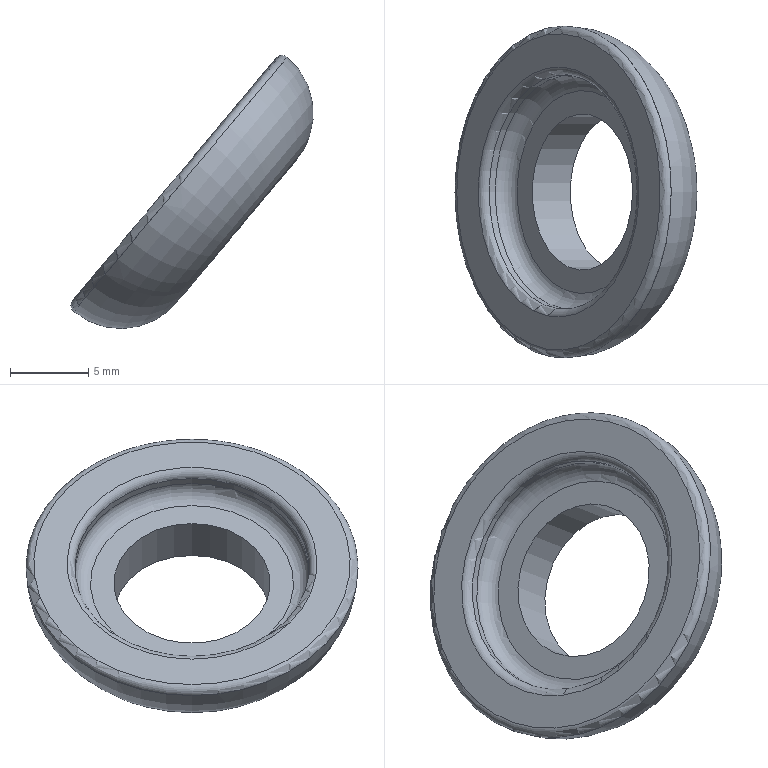Component | NX | HANGERWASHER_2 | 1 solid | 10 faces | box 15.51 x 21.25 x 17.49 mm | volume 954 mm3 | torus 4 | plane 3 | cylinder 3 | commonest cylinder face diameters 15 x1 21.25 x1 10 x1
STEP:
#1=CARTESIAN_POINT('',(0.,0.,0.));
#2=DIRECTION('',(0.,0.,1.));
#3=DIRECTION('',(1.,0.,0.));
#4=AXIS2_PLACEMENT_3D('',#1,#2,#3);
#5=CARTESIAN_POINT('',(452.874,0.,-59.196));
#6=VERTEX_POINT('',#5);
#7=CARTESIAN_POINT('',(449.66,0.,-63.026));
#8=DIRECTION('',(-0.766,0.,0.6428));
#9=DIRECTION('',(0.6428,0.,0.766));
#10=AXIS2_PLACEMENT_3D('',#7,#8,#9);
#11=CIRCLE('',#10,5.);
#12=CARTESIAN_POINT('',(449.66,0.,-63.026));
#13=DIRECTION('',(0.766,0.,-0.6428));
#14=DIRECTION('',(-0.6428,0.,-0.766));
#15=AXIS2_PLACEMENT_3D('',#12,#13,#14);
#16=PLANE('',#15);
#17=CARTESIAN_POINT('',(-5.,0.));
#18=CARTESIAN_POINT('',(-5.,8.66));
#19=CARTESIAN_POINT('',(2.5,4.33));
#20=CARTESIAN_POINT('',(10.,0.));
#21=CARTESIAN_POINT('',(2.5,-4.33));
#22=CARTESIAN_POINT('',(-5.,-8.66));
#23=CARTESIAN_POINT('',(-5.,0.));
#24=(BOUNDED_CURVE()B_SPLINE_CURVE(2,(#17,#18,#19,#20,#21,#22,#23),.UNSPECIFIED.,.T.,.F.)B_SPLINE_CURVE_WITH_KNOTS((1,2,2,2,2,1),(-2.094,0.,2.094,4.189,6.283,8.378),.UNSPECIFIED.)CURVE()GEOMETRIC_REPRESENTATION_ITEM()RATIONAL_B_SPLINE_CURVE((1.,0.5,1.,0.5,1.,0.5,1.))REPRESENTATION_ITEM(''));
#25=(GEOMETRIC_REPRESENTATION_CONTEXT(2)PARAMETRIC_REPRESENTATION_CONTEXT()REPRESENTATION_CONTEXT('',''));
#26=DEFINITIONAL_REPRESENTATION('',(#24),#25);
#27=PCURVE('',#16,#26);
#28=CARTESIAN_POINT('',(449.66,0.,-63.026));
#29=DIRECTION('',(-0.766,0.,0.6428));
#30=DIRECTION('',(0.6428,0.,0.766));
#31=AXIS2_PLACEMENT_3D('',#28,#29,#30);
#32=CYLINDRICAL_SURFACE('',#31,5.);
#33=CARTESIAN_POINT('',(0.,0.));
#34=DIRECTION('',(1.,0.));
#35=VECTOR('',#34,1.);
#36=LINE('',#33,#35);
#37=(GEOMETRIC_REPRESENTATION_CONTEXT(2)PARAMETRIC_REPRESENTATION_CONTEXT()REPRESENTATION_CONTEXT('',''));
#38=DEFINITIONAL_REPRESENTATION('',(#36),#37);
#39=PCURVE('',#32,#38);
#40=SURFACE_CURVE('',#11,(#27,#39),.PCURVE_S1.);
#41=EDGE_CURVE('',#6,#6,#40,.T.);
#42=ORIENTED_EDGE('',*,*,#41,.T.);
#43=EDGE_LOOP('',(#42));
#44=FACE_BOUND('',#43,.T.);
#45=CARTESIAN_POINT('',(445.832,0.,-67.588));
#46=VERTEX_POINT('',#45);
#47=CARTESIAN_POINT('',(449.66,0.,-63.026));
#48=DIRECTION('',(0.766,0.,-0.6428));
#49=DIRECTION('',(-0.6428,0.,-0.766));
#50=AXIS2_PLACEMENT_3D('',#47,#48,#49);
#51=CIRCLE('',#50,5.955);
#52=CARTESIAN_POINT('',(0.,0.));
#53=DIRECTION('',(1.,0.));
#54=AXIS2_PLACEMENT_2D('',#52,#53);
#55=CIRCLE('',#54,5.955);
#56=(GEOMETRIC_REPRESENTATION_CONTEXT(2)PARAMETRIC_REPRESENTATION_CONTEXT()REPRESENTATION_CONTEXT('',''));
#57=DEFINITIONAL_REPRESENTATION('',(#55),#56);
#58=PCURVE('',#16,#57);
#59=CARTESIAN_POINT('',(446.083,0.,-60.025));
#60=DIRECTION('',(0.766,0.,-0.6428));
#61=DIRECTION('',(-0.6428,0.,-0.766));
#62=AXIS2_PLACEMENT_3D('',#59,#60,#61);
#63=TOROIDAL_SURFACE('',#62,5.955,4.67);
#64=CARTESIAN_POINT('',(0.,7.854));
#65=DIRECTION('',(1.,0.));
#66=VECTOR('',#65,1.);
#67=LINE('',#64,#66);
#68=(GEOMETRIC_REPRESENTATION_CONTEXT(2)PARAMETRIC_REPRESENTATION_CONTEXT()REPRESENTATION_CONTEXT('',''));
#69=DEFINITIONAL_REPRESENTATION('',(#67),#68);
#70=PCURVE('',#63,#69);
#71=SURFACE_CURVE('',#51,(#58,#70),.PCURVE_S1.);
#72=EDGE_CURVE('',#46,#46,#71,.T.);
#73=ORIENTED_EDGE('',*,*,#72,.T.);
#74=EDGE_LOOP('',(#73));
#75=FACE_BOUND('',#74,.T.);
#76=ADVANCED_FACE('',(#44,#75),#16,.T.);
#77=CARTESIAN_POINT('',(450.9,0.,-54.276));
#78=VERTEX_POINT('',#77);
#79=CARTESIAN_POINT('',(441.258,0.,-65.767));
#80=VERTEX_POINT('',#79);
#81=CARTESIAN_POINT('',(446.079,0.,-60.021));
#82=DIRECTION('',(-0.766,0.,0.6428));
#83=DIRECTION('',(-0.6428,0.,-0.766));
#84=AXIS2_PLACEMENT_3D('',#81,#82,#83);
#85=CIRCLE('',#84,7.5);
#86=CARTESIAN_POINT('',(449.66,0.,-63.026));
#87=DIRECTION('',(-0.766,0.,0.6428));
#88=DIRECTION('',(0.6428,0.,0.766));
#89=AXIS2_PLACEMENT_3D('',#86,#87,#88);
#90=CYLINDRICAL_SURFACE('',#89,7.5);
#91=CARTESIAN_POINT('',(-3.142,4.675));
#92=DIRECTION('',(1.,0.));
#93=VECTOR('',#92,1.);
#94=LINE('',#91,#93);
#95=(GEOMETRIC_REPRESENTATION_CONTEXT(2)PARAMETRIC_REPRESENTATION_CONTEXT()REPRESENTATION_CONTEXT('',''));
#96=DEFINITIONAL_REPRESENTATION('',(#94),#95);
#97=PCURVE('',#90,#96);
#98=CARTESIAN_POINT('',(446.079,0.,-60.021));
#99=DIRECTION('',(0.766,0.,-0.6428));
#100=DIRECTION('',(-0.6428,0.,-0.766));
#101=AXIS2_PLACEMENT_3D('',#98,#99,#100);
#102=TOROIDAL_SURFACE('',#101,8.,0.5);
#103=CARTESIAN_POINT('',(6.283,3.142));
#104=DIRECTION('',(-1.,0.));
#105=VECTOR('',#104,1.);
#106=LINE('',#103,#105);
#107=(GEOMETRIC_REPRESENTATION_CONTEXT(2)PARAMETRIC_REPRESENTATION_CONTEXT()REPRESENTATION_CONTEXT('',''));
#108=DEFINITIONAL_REPRESENTATION('',(#106),#107);
#109=PCURVE('',#102,#108);
#110=SURFACE_CURVE('',#85,(#97,#109),.PCURVE_S1.);
#111=EDGE_CURVE('',#78,#80,#110,.T.);
#112=ORIENTED_EDGE('',*,*,#111,.F.);
#113=CARTESIAN_POINT('',(451.283,0.,-54.597));
#114=VERTEX_POINT('',#113);
#115=CARTESIAN_POINT('',(451.283,-0.,-54.597));
#116=CARTESIAN_POINT('',(450.9,-0.,-54.276));
#117=B_SPLINE_CURVE_WITH_KNOTS('',1,(#115,#116),.UNSPECIFIED.,.F.,.F.,(2,2),(4.175,4.675),.PIECEWISE_BEZIER_KNOTS.);
#118=CARTESIAN_POINT('',(0.,0.));
#119=DIRECTION('',(0.,1.));
#120=VECTOR('',#119,1.);
#121=LINE('',#118,#120);
#122=(GEOMETRIC_REPRESENTATION_CONTEXT(2)PARAMETRIC_REPRESENTATION_CONTEXT()REPRESENTATION_CONTEXT('',''));
#123=DEFINITIONAL_REPRESENTATION('',(#121),#122);
#124=PCURVE('',#90,#123);
#125=CARTESIAN_POINT('',(6.283,0.));
#126=DIRECTION('',(0.,1.));
#127=VECTOR('',#126,1.);
#128=LINE('',#125,#127);
#129=(GEOMETRIC_REPRESENTATION_CONTEXT(2)PARAMETRIC_REPRESENTATION_CONTEXT()REPRESENTATION_CONTEXT('',''));
#130=DEFINITIONAL_REPRESENTATION('',(#128),#129);
#131=PCURVE('',#90,#130);
#132=SEAM_CURVE('',#117,(#124,#131),.PCURVE_S1.);
#133=EDGE_CURVE('',#114,#78,#132,.T.);
#134=ORIENTED_EDGE('',*,*,#133,.F.);
#135=CARTESIAN_POINT('',(446.462,0.,-60.343));
#136=DIRECTION('',(0.766,0.,-0.6428));
#137=DIRECTION('',(0.6428,0.,0.766));
#138=AXIS2_PLACEMENT_3D('',#135,#136,#137);
#139=CIRCLE('',#138,7.5);
#140=CARTESIAN_POINT('',(6.283,4.175));
#141=DIRECTION('',(-1.,0.));
#142=VECTOR('',#141,1.);
#143=LINE('',#140,#142);
#144=(GEOMETRIC_REPRESENTATION_CONTEXT(2)PARAMETRIC_REPRESENTATION_CONTEXT()REPRESENTATION_CONTEXT('',''));
#145=DEFINITIONAL_REPRESENTATION('',(#143),#144);
#146=PCURVE('',#90,#145);
#147=CARTESIAN_POINT('',(446.462,0.,-60.343));
#148=DIRECTION('',(-0.766,0.,0.6428));
#149=DIRECTION('',(0.6428,0.,0.766));
#150=AXIS2_PLACEMENT_3D('',#147,#148,#149);
#151=TOROIDAL_SURFACE('',#150,6.5,1.);
#152=CARTESIAN_POINT('',(6.283,6.283));
#153=DIRECTION('',(-1.,0.));
#154=VECTOR('',#153,1.);
#155=LINE('',#152,#154);
#156=(GEOMETRIC_REPRESENTATION_CONTEXT(2)PARAMETRIC_REPRESENTATION_CONTEXT()REPRESENTATION_CONTEXT('',''));
#157=DEFINITIONAL_REPRESENTATION('',(#155),#156);
#158=PCURVE('',#151,#157);
#159=SURFACE_CURVE('',#139,(#146,#158),.PCURVE_S1.);
#160=EDGE_CURVE('',#114,#114,#159,.T.);
#161=ORIENTED_EDGE('',*,*,#160,.F.);
#162=ORIENTED_EDGE('',*,*,#133,.T.);
#163=CARTESIAN_POINT('',(446.079,0.,-60.021));
#164=DIRECTION('',(-0.766,0.,0.6428));
#165=DIRECTION('',(-0.6428,0.,-0.766));
#166=AXIS2_PLACEMENT_3D('',#163,#164,#165);
#167=CIRCLE('',#166,7.5);
#168=CARTESIAN_POINT('',(3.142,4.675));
#169=DIRECTION('',(1.,0.));
#170=VECTOR('',#169,1.);
#171=LINE('',#168,#170);
#172=(GEOMETRIC_REPRESENTATION_CONTEXT(2)PARAMETRIC_REPRESENTATION_CONTEXT()REPRESENTATION_CONTEXT('',''));
#173=DEFINITIONAL_REPRESENTATION('',(#171),#172);
#174=PCURVE('',#90,#173);
#175=CARTESIAN_POINT('',(6.283,3.142));
#176=DIRECTION('',(-1.,-0.));
#177=VECTOR('',#176,1.);
#178=LINE('',#175,#177);
#179=(GEOMETRIC_REPRESENTATION_CONTEXT(2)PARAMETRIC_REPRESENTATION_CONTEXT()REPRESENTATION_CONTEXT('',''));
#180=DEFINITIONAL_REPRESENTATION('',(#178),#179);
#181=PCURVE('',#102,#180);
#182=SURFACE_CURVE('',#167,(#174,#181),.PCURVE_S1.);
#183=EDGE_CURVE('',#80,#78,#182,.T.);
#184=ORIENTED_EDGE('',*,*,#183,.F.);
#185=EDGE_LOOP('',(#112,#134,#161,#162,#184));
#186=FACE_BOUND('',#185,.F.);
#187=ADVANCED_FACE('',(#186),#90,.F.);
#188=CARTESIAN_POINT('',(439.249,0.,-68.161));
#189=VERTEX_POINT('',#188);
#190=CARTESIAN_POINT('',(446.079,0.,-60.021));
#191=DIRECTION('',(0.766,0.,-0.6428));
#192=DIRECTION('',(-0.6428,0.,-0.766));
#193=AXIS2_PLACEMENT_3D('',#190,#191,#192);
#194=CIRCLE('',#193,10.625);
#195=CARTESIAN_POINT('',(449.66,0.,-63.026));
#196=DIRECTION('',(-0.766,0.,0.6428));
#197=DIRECTION('',(0.6428,0.,0.766));
#198=AXIS2_PLACEMENT_3D('',#195,#196,#197);
#199=CYLINDRICAL_SURFACE('',#198,10.625);
#200=CARTESIAN_POINT('',(9.425,4.675));
#201=DIRECTION('',(-1.,0.));
#202=VECTOR('',#201,1.);
#203=LINE('',#200,#202);
#204=(GEOMETRIC_REPRESENTATION_CONTEXT(2)PARAMETRIC_REPRESENTATION_CONTEXT()REPRESENTATION_CONTEXT('',''));
#205=DEFINITIONAL_REPRESENTATION('',(#203),#204);
#206=PCURVE('',#199,#205);
#207=CARTESIAN_POINT('',(446.079,0.,-60.021));
#208=DIRECTION('',(0.766,0.,-0.6428));
#209=DIRECTION('',(-0.6428,0.,-0.766));
#210=AXIS2_PLACEMENT_3D('',#207,#208,#209);
#211=TOROIDAL_SURFACE('',#210,10.125,0.5);
#212=CARTESIAN_POINT('',(0.,6.283));
#213=DIRECTION('',(1.,0.));
#214=VECTOR('',#213,1.);
#215=LINE('',#212,#214);
#216=(GEOMETRIC_REPRESENTATION_CONTEXT(2)PARAMETRIC_REPRESENTATION_CONTEXT()REPRESENTATION_CONTEXT('',''));
#217=DEFINITIONAL_REPRESENTATION('',(#215),#216);
#218=PCURVE('',#211,#217);
#219=SURFACE_CURVE('',#194,(#206,#218),.PCURVE_S1.);
#220=EDGE_CURVE('',#189,#189,#219,.T.);
#221=ORIENTED_EDGE('',*,*,#220,.T.);
#222=CARTESIAN_POINT('',(439.253,0.,-68.164));
#223=VERTEX_POINT('',#222);
#224=CARTESIAN_POINT('',(439.253,0.,-68.164));
#225=CARTESIAN_POINT('',(439.249,0.,-68.161));
#226=B_SPLINE_CURVE_WITH_KNOTS('',1,(#224,#225),.UNSPECIFIED.,.F.,.F.,(2,2),(4.67,4.675),.PIECEWISE_BEZIER_KNOTS.);
#227=CARTESIAN_POINT('',(3.142,0.));
#228=DIRECTION('',(0.,1.));
#229=VECTOR('',#228,1.);
#230=LINE('',#227,#229);
#231=(GEOMETRIC_REPRESENTATION_CONTEXT(2)PARAMETRIC_REPRESENTATION_CONTEXT()REPRESENTATION_CONTEXT('',''));
#232=DEFINITIONAL_REPRESENTATION('',(#230),#231);
#233=PCURVE('',#199,#232);
#234=CARTESIAN_POINT('',(9.425,0.));
#235=DIRECTION('',(0.,1.));
#236=VECTOR('',#235,1.);
#237=LINE('',#234,#236);
#238=(GEOMETRIC_REPRESENTATION_CONTEXT(2)PARAMETRIC_REPRESENTATION_CONTEXT()REPRESENTATION_CONTEXT('',''));
#239=DEFINITIONAL_REPRESENTATION('',(#237),#238);
#240=PCURVE('',#199,#239);
#241=SEAM_CURVE('',#226,(#233,#240),.PCURVE_S1.);
#242=EDGE_CURVE('',#223,#189,#241,.T.);
#243=ORIENTED_EDGE('',*,*,#242,.F.);
#244=CARTESIAN_POINT('',(446.083,0.,-60.025));
#245=DIRECTION('',(-0.766,0.,0.6428));
#246=DIRECTION('',(-0.6428,0.,-0.766));
#247=AXIS2_PLACEMENT_3D('',#244,#245,#246);
#248=CIRCLE('',#247,10.625);
#249=CARTESIAN_POINT('',(3.142,4.67));
#250=DIRECTION('',(1.,0.));
#251=VECTOR('',#250,1.);
#252=LINE('',#249,#251);
#253=(GEOMETRIC_REPRESENTATION_CONTEXT(2)PARAMETRIC_REPRESENTATION_CONTEXT()REPRESENTATION_CONTEXT('',''));
#254=DEFINITIONAL_REPRESENTATION('',(#252),#253);
#255=PCURVE('',#199,#254);
#256=CARTESIAN_POINT('',(6.283,6.283));
#257=DIRECTION('',(-1.,0.));
#258=VECTOR('',#257,1.);
#259=LINE('',#256,#258);
#260=(GEOMETRIC_REPRESENTATION_CONTEXT(2)PARAMETRIC_REPRESENTATION_CONTEXT()REPRESENTATION_CONTEXT('',''));
#261=DEFINITIONAL_REPRESENTATION('',(#259),#260);
#262=PCURVE('',#63,#261);
#263=SURFACE_CURVE('',#248,(#255,#262),.PCURVE_S1.);
#264=EDGE_CURVE('',#223,#223,#263,.T.);
#265=ORIENTED_EDGE('',*,*,#264,.T.);
#266=ORIENTED_EDGE('',*,*,#242,.T.);
#267=EDGE_LOOP('',(#221,#243,#265,#266));
#268=FACE_BOUND('',#267,.T.);
#269=ADVANCED_FACE('',(#268),#199,.T.);
#270=CARTESIAN_POINT('',(439.188,0.,-67.456));
#271=VERTEX_POINT('',#270);
#272=CARTESIAN_POINT('',(445.696,0.,-59.7));
#273=DIRECTION('',(-0.766,0.,0.6428));
#274=DIRECTION('',(-0.6428,0.,-0.766));
#275=AXIS2_PLACEMENT_3D('',#272,#273,#274);
#276=CIRCLE('',#275,10.125);
#277=CARTESIAN_POINT('',(438.866,0.,-67.839));
#278=DIRECTION('',(0.766,0.,-0.6428));
#279=DIRECTION('',(-0.6428,0.,-0.766));
#280=AXIS2_PLACEMENT_3D('',#277,#278,#279);
#281=PLANE('',#280);
#282=CARTESIAN_POINT('',(-0.5,0.));
#283=CARTESIAN_POINT('',(-0.5,-17.537));
#284=CARTESIAN_POINT('',(-15.688,-8.769));
#285=CARTESIAN_POINT('',(-30.875,-0.));
#286=CARTESIAN_POINT('',(-15.688,8.769));
#287=CARTESIAN_POINT('',(-0.5,17.537));
#288=CARTESIAN_POINT('',(-0.5,0.));
#289=(BOUNDED_CURVE()B_SPLINE_CURVE(2,(#282,#283,#284,#285,#286,#287,#288),.UNSPECIFIED.,.T.,.F.)B_SPLINE_CURVE_WITH_KNOTS((1,2,2,2,2,1),(-2.094,0.,2.094,4.189,6.283,8.378),.UNSPECIFIED.)CURVE()GEOMETRIC_REPRESENTATION_ITEM()RATIONAL_B_SPLINE_CURVE((1.,0.5,1.,0.5,1.,0.5,1.))REPRESENTATION_ITEM(''));
#290=(GEOMETRIC_REPRESENTATION_CONTEXT(2)PARAMETRIC_REPRESENTATION_CONTEXT()REPRESENTATION_CONTEXT('',''));
#291=DEFINITIONAL_REPRESENTATION('',(#289),#290);
#292=PCURVE('',#281,#291);
#293=CARTESIAN_POINT('',(6.283,4.712));
#294=DIRECTION('',(-1.,0.));
#295=VECTOR('',#294,1.);
#296=LINE('',#293,#295);
#297=(GEOMETRIC_REPRESENTATION_CONTEXT(2)PARAMETRIC_REPRESENTATION_CONTEXT()REPRESENTATION_CONTEXT('',''));
#298=DEFINITIONAL_REPRESENTATION('',(#296),#297);
#299=PCURVE('',#211,#298);
#300=SURFACE_CURVE('',#276,(#292,#299),.PCURVE_S1.);
#301=EDGE_CURVE('',#271,#271,#300,.T.);
#302=ORIENTED_EDGE('',*,*,#301,.T.);
#303=EDGE_LOOP('',(#302));
#304=FACE_BOUND('',#303,.T.);
#305=CARTESIAN_POINT('',(440.554,0.,-65.828));
#306=VERTEX_POINT('',#305);
#307=CARTESIAN_POINT('',(445.696,0.,-59.7));
#308=DIRECTION('',(0.766,0.,-0.6428));
#309=DIRECTION('',(-0.6428,0.,-0.766));
#310=AXIS2_PLACEMENT_3D('',#307,#308,#309);
#311=CIRCLE('',#310,8.);
#312=CARTESIAN_POINT('',(-10.625,0.));
#313=DIRECTION('',(1.,0.));
#314=AXIS2_PLACEMENT_2D('',#312,#313);
#315=CIRCLE('',#314,8.);
#316=(GEOMETRIC_REPRESENTATION_CONTEXT(2)PARAMETRIC_REPRESENTATION_CONTEXT()REPRESENTATION_CONTEXT('',''));
#317=DEFINITIONAL_REPRESENTATION('',(#315),#316);
#318=PCURVE('',#281,#317);
#319=CARTESIAN_POINT('',(0.,4.712));
#320=DIRECTION('',(1.,0.));
#321=VECTOR('',#320,1.);
#322=LINE('',#319,#321);
#323=(GEOMETRIC_REPRESENTATION_CONTEXT(2)PARAMETRIC_REPRESENTATION_CONTEXT()REPRESENTATION_CONTEXT('',''));
#324=DEFINITIONAL_REPRESENTATION('',(#322),#323);
#325=PCURVE('',#102,#324);
#326=SURFACE_CURVE('',#311,(#318,#325),.PCURVE_S1.);
#327=EDGE_CURVE('',#306,#306,#326,.T.);
#328=ORIENTED_EDGE('',*,*,#327,.T.);
#329=EDGE_LOOP('',(#328));
#330=FACE_BOUND('',#329,.T.);
#331=ADVANCED_FACE('',(#304,#330),#281,.F.);
#332=CARTESIAN_POINT('',(450.442,0.,-57.155));
#333=VERTEX_POINT('',#332);
#334=CARTESIAN_POINT('',(447.228,0.,-60.986));
#335=DIRECTION('',(-0.766,0.,0.6428));
#336=DIRECTION('',(0.6428,0.,0.766));
#337=AXIS2_PLACEMENT_3D('',#334,#335,#336);
#338=CIRCLE('',#337,5.);
#339=CARTESIAN_POINT('',(447.228,0.,-60.986));
#340=DIRECTION('',(-0.766,0.,0.6428));
#341=DIRECTION('',(0.6428,0.,0.766));
#342=AXIS2_PLACEMENT_3D('',#339,#340,#341);
#343=PLANE('',#342);
#344=CARTESIAN_POINT('',(0.,0.));
#345=DIRECTION('',(1.,0.));
#346=AXIS2_PLACEMENT_2D('',#344,#345);
#347=CIRCLE('',#346,5.);
#348=(GEOMETRIC_REPRESENTATION_CONTEXT(2)PARAMETRIC_REPRESENTATION_CONTEXT()REPRESENTATION_CONTEXT('',''));
#349=DEFINITIONAL_REPRESENTATION('',(#347),#348);
#350=PCURVE('',#343,#349);
#351=CARTESIAN_POINT('',(0.,3.175));
#352=DIRECTION('',(1.,0.));
#353=VECTOR('',#352,1.);
#354=LINE('',#351,#353);
#355=(GEOMETRIC_REPRESENTATION_CONTEXT(2)PARAMETRIC_REPRESENTATION_CONTEXT()REPRESENTATION_CONTEXT('',''));
#356=DEFINITIONAL_REPRESENTATION('',(#354),#355);
#357=PCURVE('',#32,#356);
#358=SURFACE_CURVE('',#338,(#350,#357),.PCURVE_S1.);
#359=EDGE_CURVE('',#333,#333,#358,.T.);
#360=ORIENTED_EDGE('',*,*,#359,.F.);
#361=EDGE_LOOP('',(#360));
#362=FACE_BOUND('',#361,.T.);
#363=CARTESIAN_POINT('',(451.406,0.,-56.006));
#364=VERTEX_POINT('',#363);
#365=CARTESIAN_POINT('',(447.228,0.,-60.986));
#366=DIRECTION('',(-0.766,0.,0.6428));
#367=DIRECTION('',(0.6428,0.,0.766));
#368=AXIS2_PLACEMENT_3D('',#365,#366,#367);
#369=CIRCLE('',#368,6.5);
#370=CARTESIAN_POINT('',(0.,0.));
#371=DIRECTION('',(1.,0.));
#372=AXIS2_PLACEMENT_2D('',#370,#371);
#373=CIRCLE('',#372,6.5);
#374=(GEOMETRIC_REPRESENTATION_CONTEXT(2)PARAMETRIC_REPRESENTATION_CONTEXT()REPRESENTATION_CONTEXT('',''));
#375=DEFINITIONAL_REPRESENTATION('',(#373),#374);
#376=PCURVE('',#343,#375);
#377=CARTESIAN_POINT('',(0.,4.712));
#378=DIRECTION('',(1.,0.));
#379=VECTOR('',#378,1.);
#380=LINE('',#377,#379);
#381=(GEOMETRIC_REPRESENTATION_CONTEXT(2)PARAMETRIC_REPRESENTATION_CONTEXT()REPRESENTATION_CONTEXT('',''));
#382=DEFINITIONAL_REPRESENTATION('',(#380),#381);
#383=PCURVE('',#151,#382);
#384=SURFACE_CURVE('',#369,(#376,#383),.PCURVE_S1.);
#385=EDGE_CURVE('',#364,#364,#384,.T.);
#386=ORIENTED_EDGE('',*,*,#385,.T.);
#387=EDGE_LOOP('',(#386));
#388=FACE_BOUND('',#387,.T.);
#389=ADVANCED_FACE('',(#362,#388),#343,.T.);
#390=ORIENTED_EDGE('',*,*,#220,.F.);
#391=CARTESIAN_POINT('',(439.188,-0.,-67.456));
#392=CARTESIAN_POINT('',(439.102,-0.,-67.559));
#393=CARTESIAN_POINT('',(439.051,-0.,-67.686));
#394=CARTESIAN_POINT('',(439.041,-0.,-67.824));
#395=CARTESIAN_POINT('',(439.074,-0.,-67.958));
#396=CARTESIAN_POINT('',(439.147,-0.,-68.075));
#397=CARTESIAN_POINT('',(439.249,-0.,-68.161));
#398=(BOUNDED_CURVE()B_SPLINE_CURVE(6,(#391,#392,#393,#394,#395,#396,#397),.UNSPECIFIED.,.F.,.F.)B_SPLINE_CURVE_WITH_KNOTS((7,7),(-1.571,0.),.PIECEWISE_BEZIER_KNOTS.)CURVE()GEOMETRIC_REPRESENTATION_ITEM()RATIONAL_B_SPLINE_CURVE((1.031,1.01,0.9979,0.994,0.9979,1.01,1.031))REPRESENTATION_ITEM(''));
#399=CARTESIAN_POINT('',(0.,6.283));
#400=DIRECTION('',(0.,1.));
#401=VECTOR('',#400,1.);
#402=LINE('',#399,#401);
#403=(GEOMETRIC_REPRESENTATION_CONTEXT(2)PARAMETRIC_REPRESENTATION_CONTEXT()REPRESENTATION_CONTEXT('',''));
#404=DEFINITIONAL_REPRESENTATION('',(#402),#403);
#405=PCURVE('',#211,#404);
#406=CARTESIAN_POINT('',(6.283,6.283));
#407=DIRECTION('',(0.,1.));
#408=VECTOR('',#407,1.);
#409=LINE('',#406,#408);
#410=(GEOMETRIC_REPRESENTATION_CONTEXT(2)PARAMETRIC_REPRESENTATION_CONTEXT()REPRESENTATION_CONTEXT('',''));
#411=DEFINITIONAL_REPRESENTATION('',(#409),#410);
#412=PCURVE('',#211,#411);
#413=SEAM_CURVE('',#398,(#405,#412),.PCURVE_S1.);
#414=EDGE_CURVE('',#271,#189,#413,.T.);
#415=ORIENTED_EDGE('',*,*,#414,.F.);
#416=ORIENTED_EDGE('',*,*,#301,.F.);
#417=ORIENTED_EDGE('',*,*,#414,.T.);
#418=EDGE_LOOP('',(#390,#415,#416,#417));
#419=FACE_BOUND('',#418,.T.);
#420=ADVANCED_FACE('',(#419),#211,.T.);
#421=ORIENTED_EDGE('',*,*,#327,.F.);
#422=CARTESIAN_POINT('',(441.258,-0.,-65.767));
#423=CARTESIAN_POINT('',(441.156,-0.,-65.681));
#424=CARTESIAN_POINT('',(441.029,-0.,-65.63));
#425=CARTESIAN_POINT('',(440.89,-0.,-65.62));
#426=CARTESIAN_POINT('',(440.756,-0.,-65.654));
#427=CARTESIAN_POINT('',(440.64,-0.,-65.726));
#428=CARTESIAN_POINT('',(440.554,-0.,-65.828));
#429=(BOUNDED_CURVE()B_SPLINE_CURVE(6,(#422,#423,#424,#425,#426,#427,#428),.UNSPECIFIED.,.F.,.F.)B_SPLINE_CURVE_WITH_KNOTS((7,7),(3.142,4.712),.PIECEWISE_BEZIER_KNOTS.)CURVE()GEOMETRIC_REPRESENTATION_ITEM()RATIONAL_B_SPLINE_CURVE((1.031,1.01,0.9979,0.994,0.9979,1.01,1.031))REPRESENTATION_ITEM(''));
#430=CARTESIAN_POINT('',(0.,0.));
#431=DIRECTION('',(0.,1.));
#432=VECTOR('',#431,1.);
#433=LINE('',#430,#432);
#434=(GEOMETRIC_REPRESENTATION_CONTEXT(2)PARAMETRIC_REPRESENTATION_CONTEXT()REPRESENTATION_CONTEXT('',''));
#435=DEFINITIONAL_REPRESENTATION('',(#433),#434);
#436=PCURVE('',#102,#435);
#437=CARTESIAN_POINT('',(6.283,0.));
#438=DIRECTION('',(0.,1.));
#439=VECTOR('',#438,1.);
#440=LINE('',#437,#439);
#441=(GEOMETRIC_REPRESENTATION_CONTEXT(2)PARAMETRIC_REPRESENTATION_CONTEXT()REPRESENTATION_CONTEXT('',''));
#442=DEFINITIONAL_REPRESENTATION('',(#440),#441);
#443=PCURVE('',#102,#442);
#444=SEAM_CURVE('',#429,(#436,#443),.PCURVE_S1.);
#445=EDGE_CURVE('',#80,#306,#444,.T.);
#446=ORIENTED_EDGE('',*,*,#445,.F.);
#447=ORIENTED_EDGE('',*,*,#111,.F.);
#448=ORIENTED_EDGE('',*,*,#183,.F.);
#449=ORIENTED_EDGE('',*,*,#445,.T.);
#450=EDGE_LOOP('',(#421,#446,#447,#448,#449));
#451=FACE_BOUND('',#450,.T.);
#452=ADVANCED_FACE('',(#451),#102,.T.);
#453=ORIENTED_EDGE('',*,*,#385,.T.);
#454=CARTESIAN_POINT('',(451.406,0.,-56.006));
#455=CARTESIAN_POINT('',(451.578,0.,-55.802));
#456=CARTESIAN_POINT('',(451.68,0.,-55.547));
#457=CARTESIAN_POINT('',(451.699,0.,-55.271));
#458=CARTESIAN_POINT('',(451.632,0.,-55.002));
#459=CARTESIAN_POINT('',(451.488,0.,-54.769));
#460=CARTESIAN_POINT('',(451.283,0.,-54.597));
#461=(BOUNDED_CURVE()B_SPLINE_CURVE(6,(#454,#455,#456,#457,#458,#459,#460),.UNSPECIFIED.,.F.,.F.)B_SPLINE_CURVE_WITH_KNOTS((7,7),(4.712,6.283),.PIECEWISE_BEZIER_KNOTS.)CURVE()GEOMETRIC_REPRESENTATION_ITEM()RATIONAL_B_SPLINE_CURVE((1.031,1.01,0.9979,0.994,0.9979,1.01,1.031))REPRESENTATION_ITEM(''));
#462=CARTESIAN_POINT('',(6.283,0.));
#463=DIRECTION('',(0.,1.));
#464=VECTOR('',#463,1.);
#465=LINE('',#462,#464);
#466=(GEOMETRIC_REPRESENTATION_CONTEXT(2)PARAMETRIC_REPRESENTATION_CONTEXT()REPRESENTATION_CONTEXT('',''));
#467=DEFINITIONAL_REPRESENTATION('',(#465),#466);
#468=PCURVE('',#151,#467);
#469=CARTESIAN_POINT('',(0.,0.));
#470=DIRECTION('',(0.,1.));
#471=VECTOR('',#470,1.);
#472=LINE('',#469,#471);
#473=(GEOMETRIC_REPRESENTATION_CONTEXT(2)PARAMETRIC_REPRESENTATION_CONTEXT()REPRESENTATION_CONTEXT('',''));
#474=DEFINITIONAL_REPRESENTATION('',(#472),#473);
#475=PCURVE('',#151,#474);
#476=SEAM_CURVE('',#461,(#468,#475),.PCURVE_S1.);
#477=EDGE_CURVE('',#364,#114,#476,.T.);
#478=ORIENTED_EDGE('',*,*,#477,.T.);
#479=ORIENTED_EDGE('',*,*,#160,.T.);
#480=ORIENTED_EDGE('',*,*,#477,.F.);
#481=EDGE_LOOP('',(#453,#478,#479,#480));
#482=FACE_BOUND('',#481,.F.);
#483=ADVANCED_FACE('',(#482),#151,.F.);
#484=ORIENTED_EDGE('',*,*,#72,.F.);
#485=CARTESIAN_POINT('',(439.253,-0.,-68.164));
#486=CARTESIAN_POINT('',(440.209,-0.,-68.966));
#487=CARTESIAN_POINT('',(441.396,-0.,-69.444));
#488=CARTESIAN_POINT('',(442.688,-0.,-69.533));
#489=CARTESIAN_POINT('',(443.944,-0.,-69.221));
#490=CARTESIAN_POINT('',(445.03,-0.,-68.545));
#491=CARTESIAN_POINT('',(445.832,-0.,-67.588));
#492=(BOUNDED_CURVE()B_SPLINE_CURVE(6,(#485,#486,#487,#488,#489,#490,#491),.UNSPECIFIED.,.F.,.F.)B_SPLINE_CURVE_WITH_KNOTS((7,7),(0.,1.571),.PIECEWISE_BEZIER_KNOTS.)CURVE()GEOMETRIC_REPRESENTATION_ITEM()RATIONAL_B_SPLINE_CURVE((1.031,1.01,0.9979,0.994,0.9979,1.01,1.031))REPRESENTATION_ITEM(''));
#493=CARTESIAN_POINT('',(0.,6.283));
#494=DIRECTION('',(0.,1.));
#495=VECTOR('',#494,1.);
#496=LINE('',#493,#495);
#497=(GEOMETRIC_REPRESENTATION_CONTEXT(2)PARAMETRIC_REPRESENTATION_CONTEXT()REPRESENTATION_CONTEXT('',''));
#498=DEFINITIONAL_REPRESENTATION('',(#496),#497);
#499=PCURVE('',#63,#498);
#500=CARTESIAN_POINT('',(6.283,6.283));
#501=DIRECTION('',(0.,1.));
#502=VECTOR('',#501,1.);
#503=LINE('',#500,#502);
#504=(GEOMETRIC_REPRESENTATION_CONTEXT(2)PARAMETRIC_REPRESENTATION_CONTEXT()REPRESENTATION_CONTEXT('',''));
#505=DEFINITIONAL_REPRESENTATION('',(#503),#504);
#506=PCURVE('',#63,#505);
#507=SEAM_CURVE('',#492,(#499,#506),.PCURVE_S1.);
#508=EDGE_CURVE('',#223,#46,#507,.T.);
#509=ORIENTED_EDGE('',*,*,#508,.F.);
#510=ORIENTED_EDGE('',*,*,#264,.F.);
#511=ORIENTED_EDGE('',*,*,#508,.T.);
#512=EDGE_LOOP('',(#484,#509,#510,#511));
#513=FACE_BOUND('',#512,.T.);
#514=ADVANCED_FACE('',(#513),#63,.T.);
#515=ORIENTED_EDGE('',*,*,#359,.F.);
#516=CARTESIAN_POINT('',(452.874,-0.,-59.196));
#517=CARTESIAN_POINT('',(450.442,-0.,-57.155));
#518=B_SPLINE_CURVE_WITH_KNOTS('',1,(#516,#517),.UNSPECIFIED.,.F.,.F.,(2,2),(0.,3.175),.PIECEWISE_BEZIER_KNOTS.);
#519=CARTESIAN_POINT('',(0.,0.));
#520=DIRECTION('',(0.,1.));
#521=VECTOR('',#520,1.);
#522=LINE('',#519,#521);
#523=(GEOMETRIC_REPRESENTATION_CONTEXT(2)PARAMETRIC_REPRESENTATION_CONTEXT()REPRESENTATION_CONTEXT('',''));
#524=DEFINITIONAL_REPRESENTATION('',(#522),#523);
#525=PCURVE('',#32,#524);
#526=CARTESIAN_POINT('',(6.283,0.));
#527=DIRECTION('',(0.,1.));
#528=VECTOR('',#527,1.);
#529=LINE('',#526,#528);
#530=(GEOMETRIC_REPRESENTATION_CONTEXT(2)PARAMETRIC_REPRESENTATION_CONTEXT()REPRESENTATION_CONTEXT('',''));
#531=DEFINITIONAL_REPRESENTATION('',(#529),#530);
#532=PCURVE('',#32,#531);
#533=SEAM_CURVE('',#518,(#525,#532),.PCURVE_S1.);
#534=EDGE_CURVE('',#6,#333,#533,.T.);
#535=ORIENTED_EDGE('',*,*,#534,.F.);
#536=ORIENTED_EDGE('',*,*,#41,.T.);
#537=ORIENTED_EDGE('',*,*,#534,.T.);
#538=EDGE_LOOP('',(#515,#535,#536,#537));
#539=FACE_BOUND('',#538,.F.);
#540=ADVANCED_FACE('',(#539),#32,.F.);
#541=CLOSED_SHELL('',(#76,#187,#269,#331,#389,#420,#452,#483,#514,#540));
#542=MANIFOLD_SOLID_BREP('',#541);
#543=(LENGTH_UNIT()NAMED_UNIT(*)SI_UNIT(.MILLI.,.METRE.));
#544=UNCERTAINTY_MEASURE_WITH_UNIT(LENGTH_MEASURE(0.00001),#543,'','');
#545=(NAMED_UNIT(*)PLANE_ANGLE_UNIT()SI_UNIT($,.RADIAN.));
#546=(NAMED_UNIT(*)SI_UNIT($,.STERADIAN.)SOLID_ANGLE_UNIT());
#547=(GEOMETRIC_REPRESENTATION_CONTEXT(3)GLOBAL_UNCERTAINTY_ASSIGNED_CONTEXT((#544))GLOBAL_UNIT_ASSIGNED_CONTEXT((#543,#545,#546))REPRESENTATION_CONTEXT('',''));
#548=ADVANCED_BREP_SHAPE_REPRESENTATION('',(#4,#542),#547);